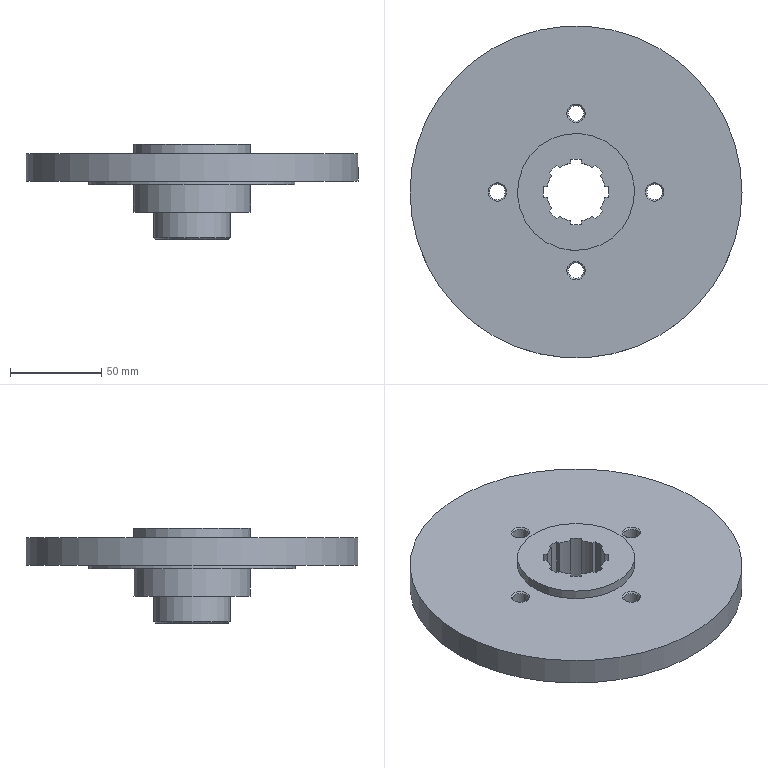Component | NX | ZYC63 | 1 solid | 56 faces | volume 442444 mm3 | cylinder 25 | plane 22 | cone 9 | commonest cylinder face diameters 32 x8 36 x8 8.5 x4 64 x2 42 x1 181.5 x1 113 x1